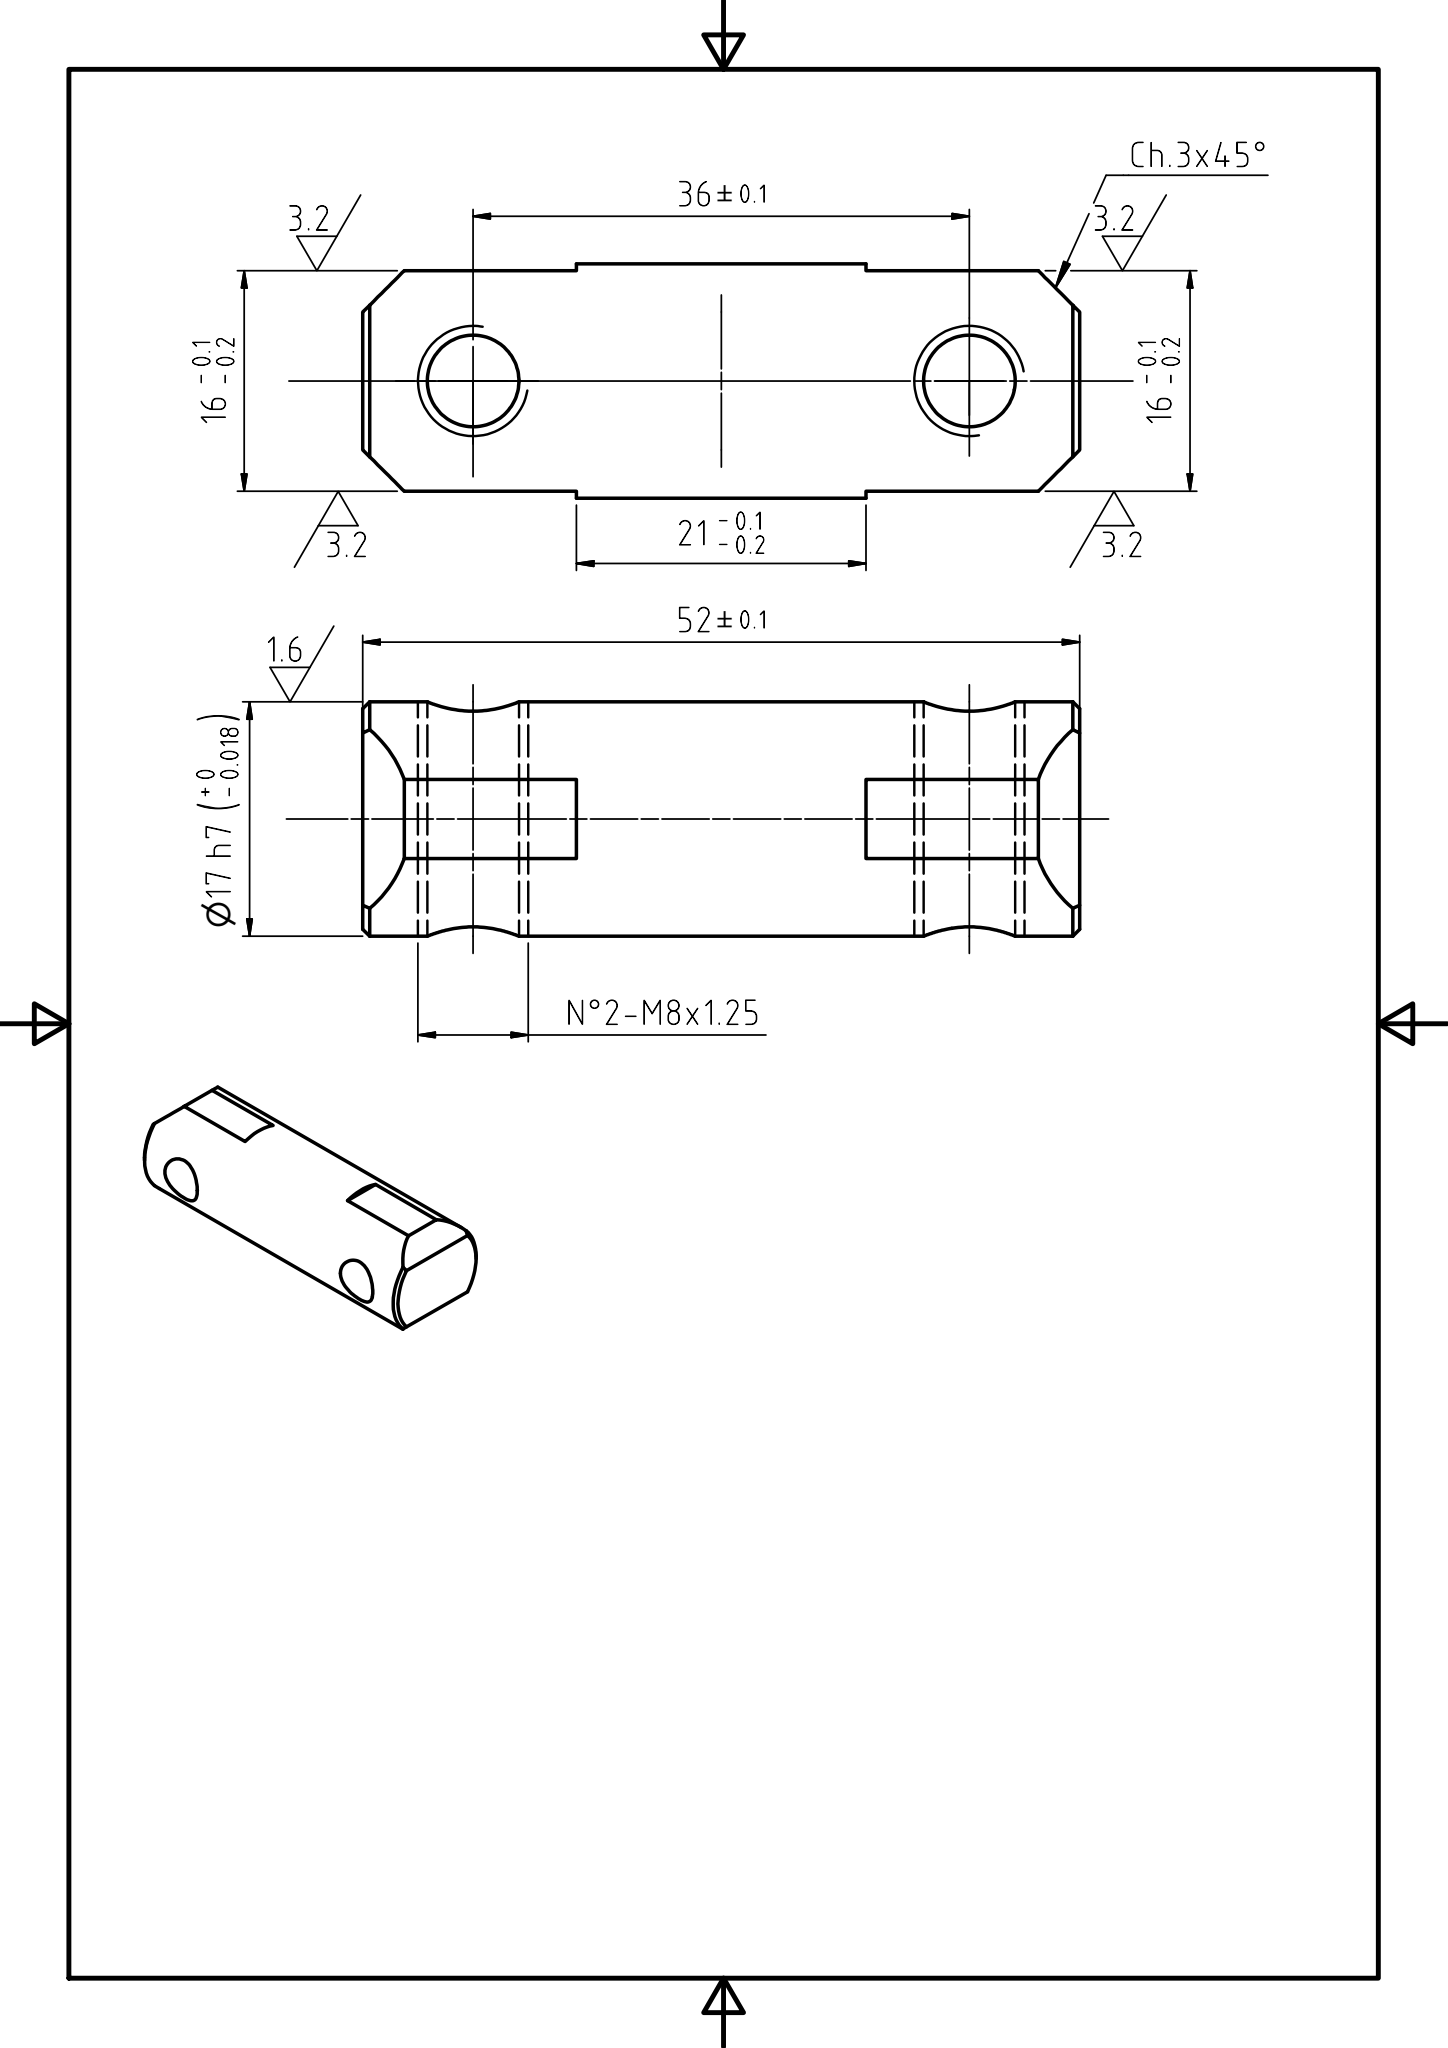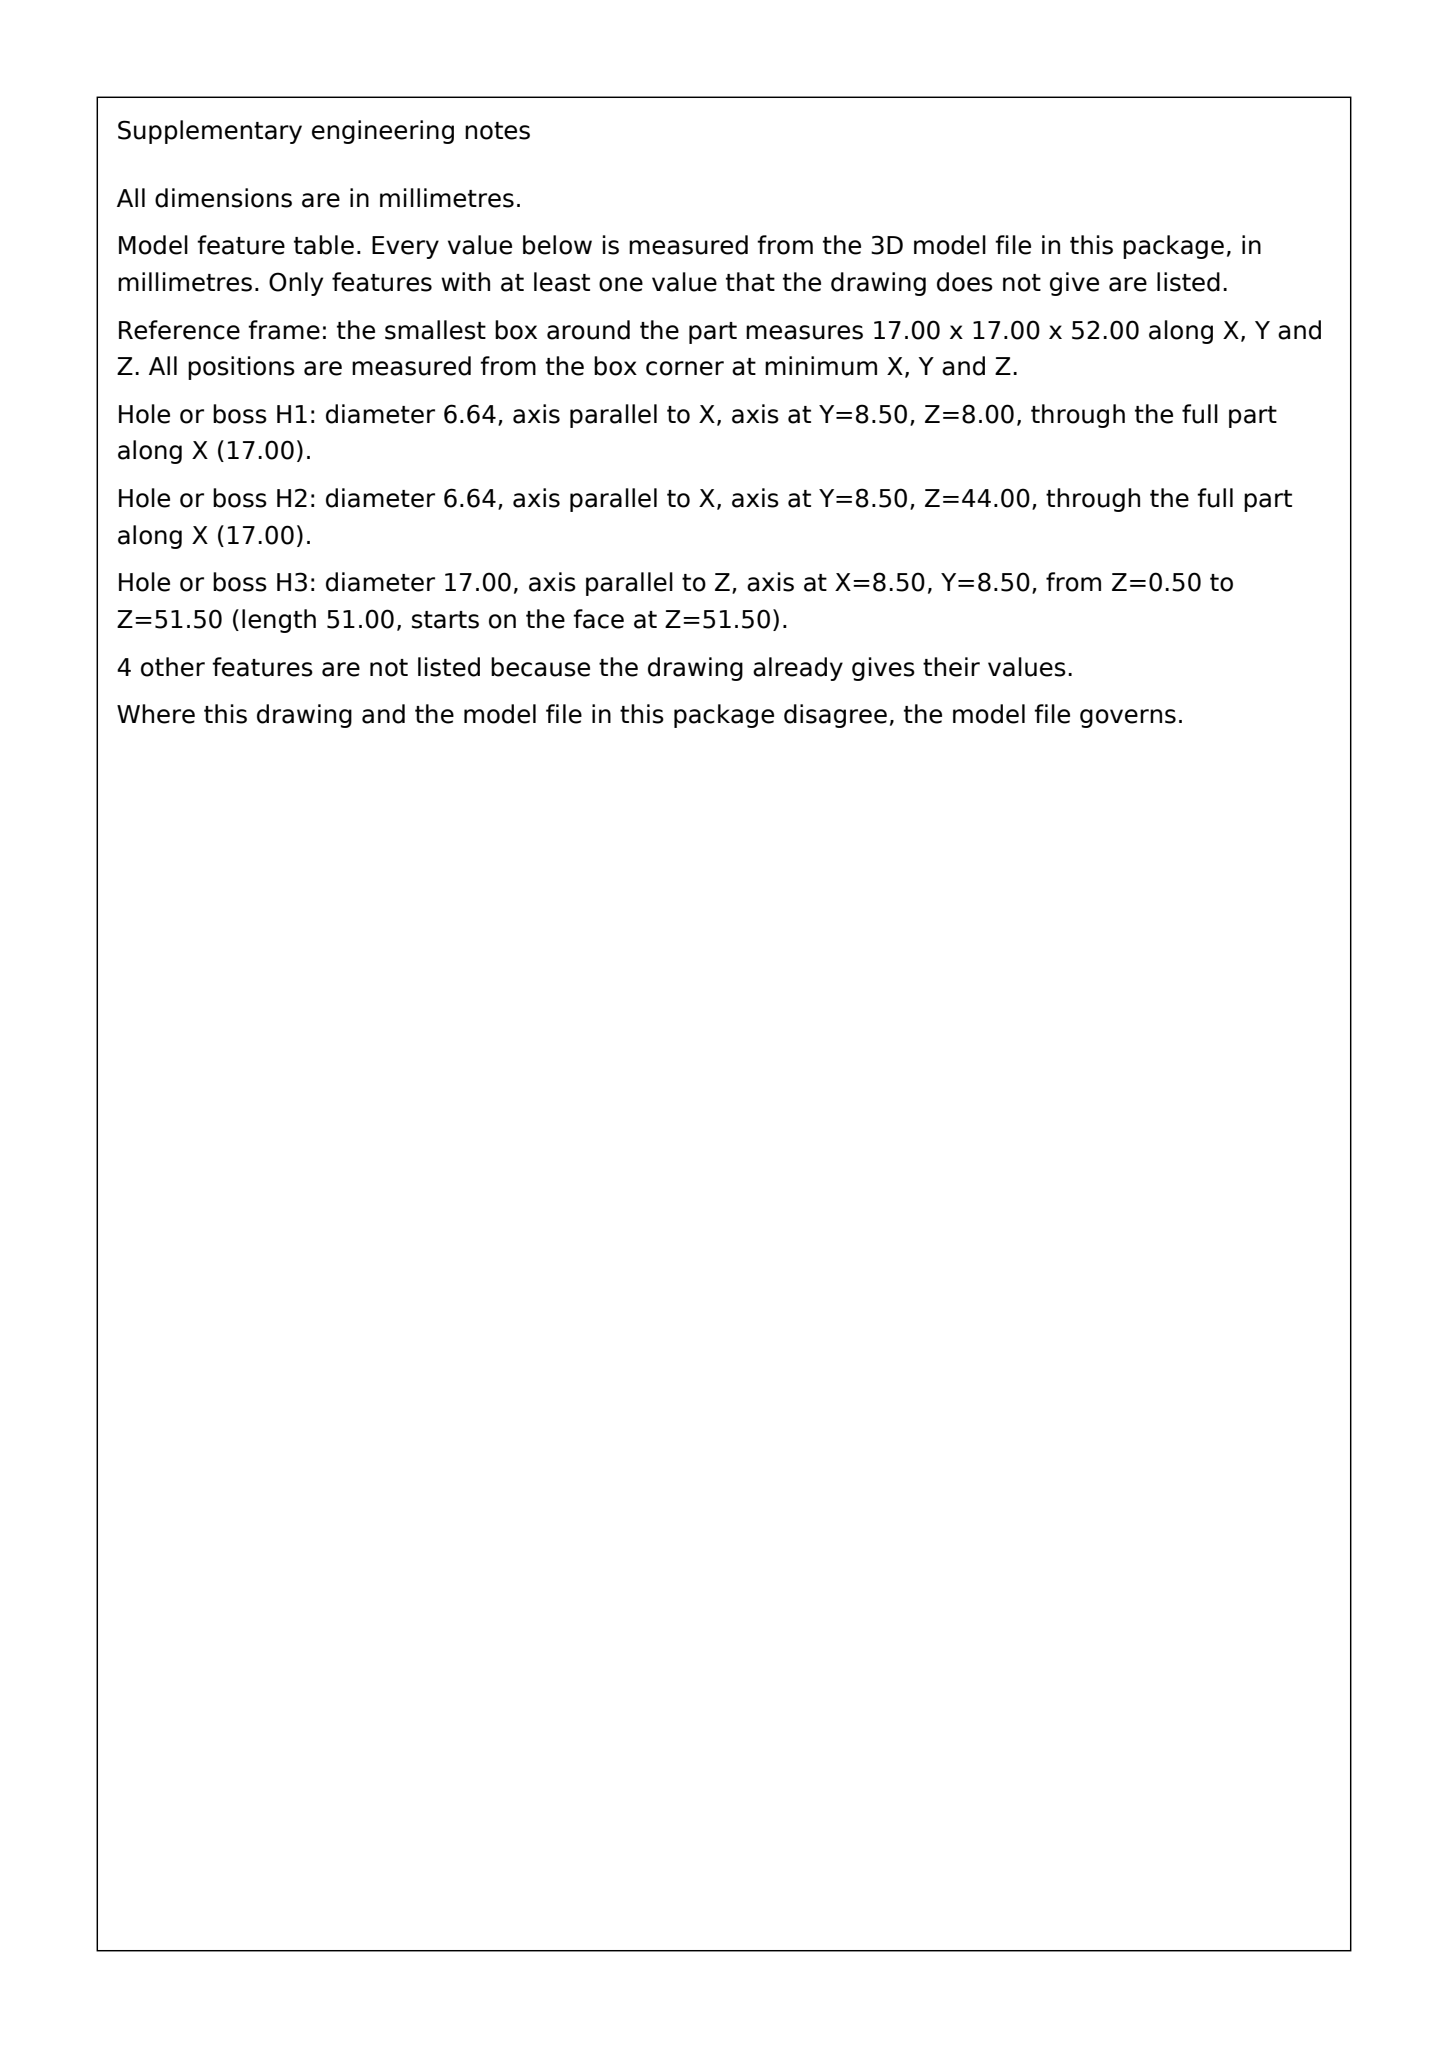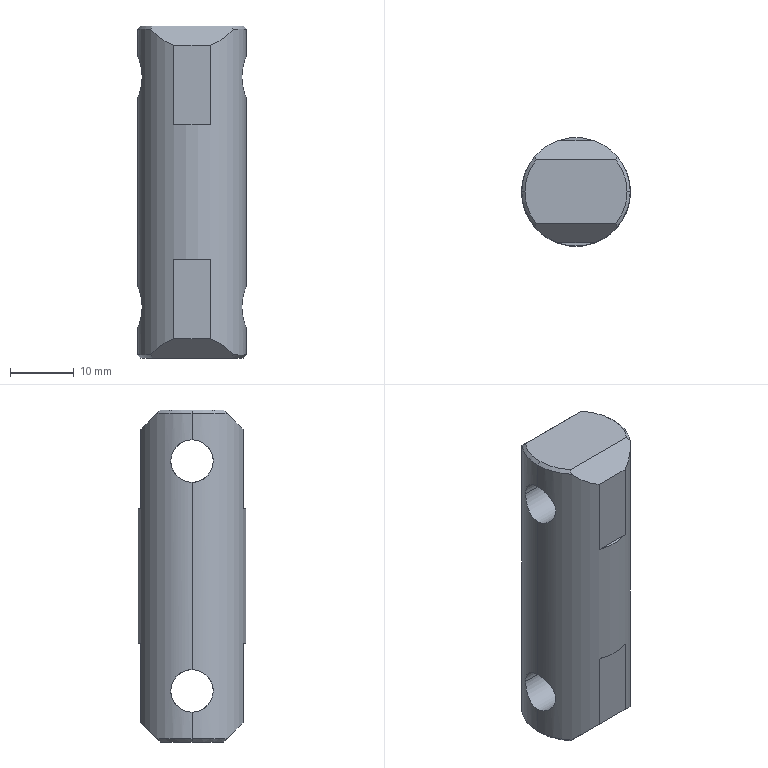Part | SolidWorks | mm | 1 solid | 28 faces | box 17 x 17 x 52 mm | volume 10353 mm3 | plane 14 | cone 8 | cylinder 6 | commonest cylinder face diameters 6.647 x4 17 x2